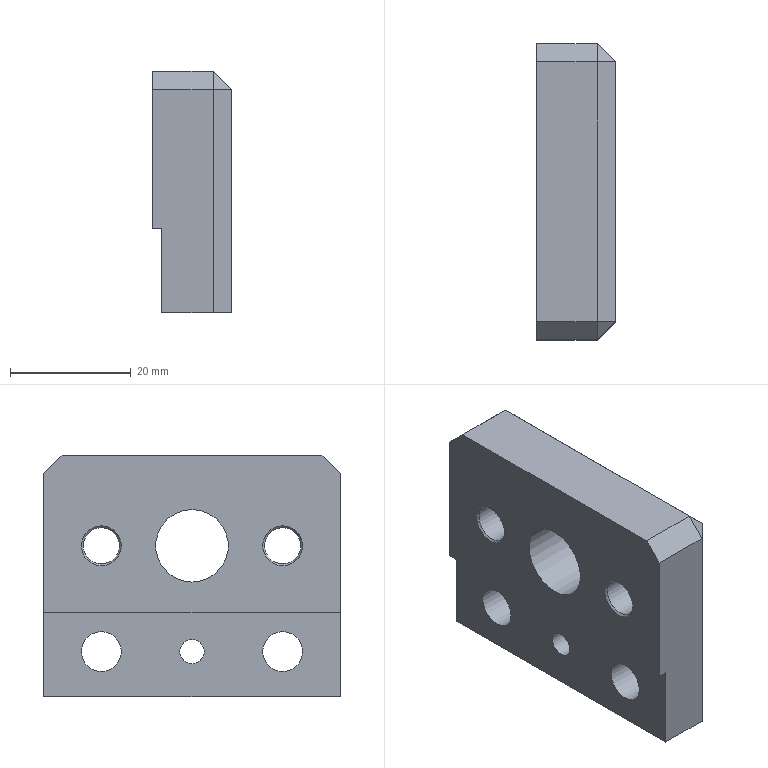Component | NX | FIXED_BRACKET | 1 solid | 27 faces | volume 19872 mm3 | plane 17 | cylinder 8 | cone 2 | commonest cylinder face diameters 6.6 x2 11 x2 6 x2 4 x1 12 x1